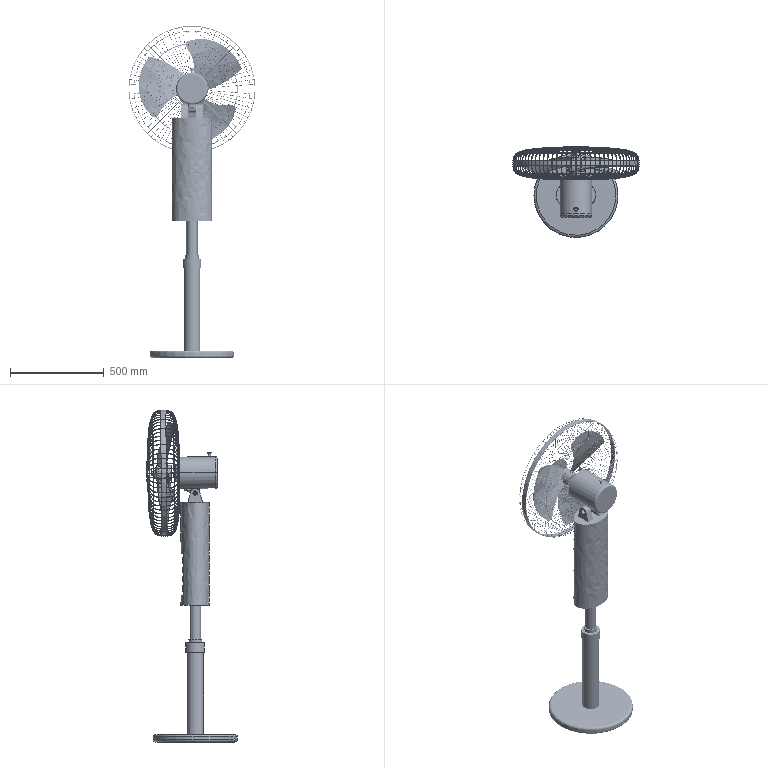Assembly | NX | mm | 15 component files | 22 solids | 1488 faces | box 678.09 x 483.76 x 1775.79 mm | volume 26298910 mm3 | cylinder 545 | plane 366 | spline 352 | torus 212 | cone 12 | other 1 | commonest cylinder face diameters 1.587 x232 1.588 x188 1 x18 75 x15 30 x10 60 x8 19.05 x6 86.6 x5
Bill of materials:
unnamed part 1 | 1 |  | Revolved part: a thin circular flange with a tapered (conical) body on one side and a short, smaller cylindrical boss on the other. There is a recessed central bore.
unnamed part 2 | 1 |  | Assembly-like body: a large, round, domed wire-mesh guard with a solid outer band. A cylindrical housing sticks out from its center on one side, and a short knob or pin sits on top of the housing. The overall shape resembles a fan guard with a motor housing.
unnamed part 3 | 1 |  | Plain solid straight cylindrical rod with flat ends.
unnamed part 4 | 1 |  | Stepped cylindrical bushing/sleeve: a larger-diameter section with a coaxial smaller-diameter collar on top, and a central bore through both.
unnamed part 5 | 1 |  | Bracket-like block: a roughly rectangular body with rounded vertical corners. A two-step cylindrical boss sits on top near one end, and a curved lug hangs below with a round through hole whose axis is perpendicular to the boss axis.
unnamed part 6 | 1 |  | Solid stepped pin/shaft: a larger-diameter cylinder joined coaxially to a smaller-diameter, shorter-length cylinder, with small edge chamfers at the ends.
unnamed part 7 | 1 |  | A cylindrical drum with rounded ends and rows of small holes on its curved wall. A thin circular flange sits around its middle, and a long slender coaxial rod extends from one end with two short, larger-diameter sleeve sections along it.
unnamed part 8 | 1 |  | Three-blade axial rotor: a small cylindrical hub with three broad, swept, twisted blades spaced evenly around it, and a small central hole in the hub.
unnamed part 9 | 4 |  | Short solid cylinder/plug, rounded or filleted around the edge of one end face; the opposite end is flat with a sharp edge.
unnamed part 10 | 1 |  | Thin flat circular disc/washer with slightly rounded outer edges. A small off-center hole is visible in the isometric view.
unnamed part 11 | 1 |  | An oval (elliptical) cylindrical body with two flat tabs sticking up from one end face. Each tab has a tapered top with a round hole. The overall form resembles a can-type component with terminal tabs.
unnamed part 12 | 1 |  | Straight cylindrical tube with a concentric bore that is open at one end.
Mates:
1. fix | upper_link_column 1 component
2. touch align | connector 1 face | upper_link_column 1 face
3. center | connector 1 face | connector 1 face | upper_link_column 1 face | upper_link_column 1 face
4. center | upper_link_column 1 face | upper_link_column 1 face | outer_cover 1 face | outer_cover 1 face
5. touch align | connector 1 face | outer_cover 1 face
6. touch align | connecting_shaft 1 face | outer_cover 1 face
7. concentric | connecting_shaft 1 edge | outer_cover 1 edge
8. concentric | snap_cover 1 edge | connecting_shaft 1 edge
9. concentric | fan_blade 1 edge | snap_cover 1 edge
10. concentric | connecting_rod 1 edge | upper_link_column 1 edge
11. concentric | lower_link_rod 1 edge | connecting_rod 1 edge
12. concentric | lower_link_rod 1 arc | connecting_sleeve 1 edge
13. concentric | lower_link_rod 1 edge | base 1 edge
14. concentric | button 4 edge | upper_link_column 1 edge
15. concentric | button 3 edge | upper_link_column 1 edge
16. concentric | button 2 edge | upper_link_column 1 edge
17. concentric | button 1 edge | upper_link_column 1 edge
18. concentric | connecting_pin 1 edge | upper_link_column 1 edge